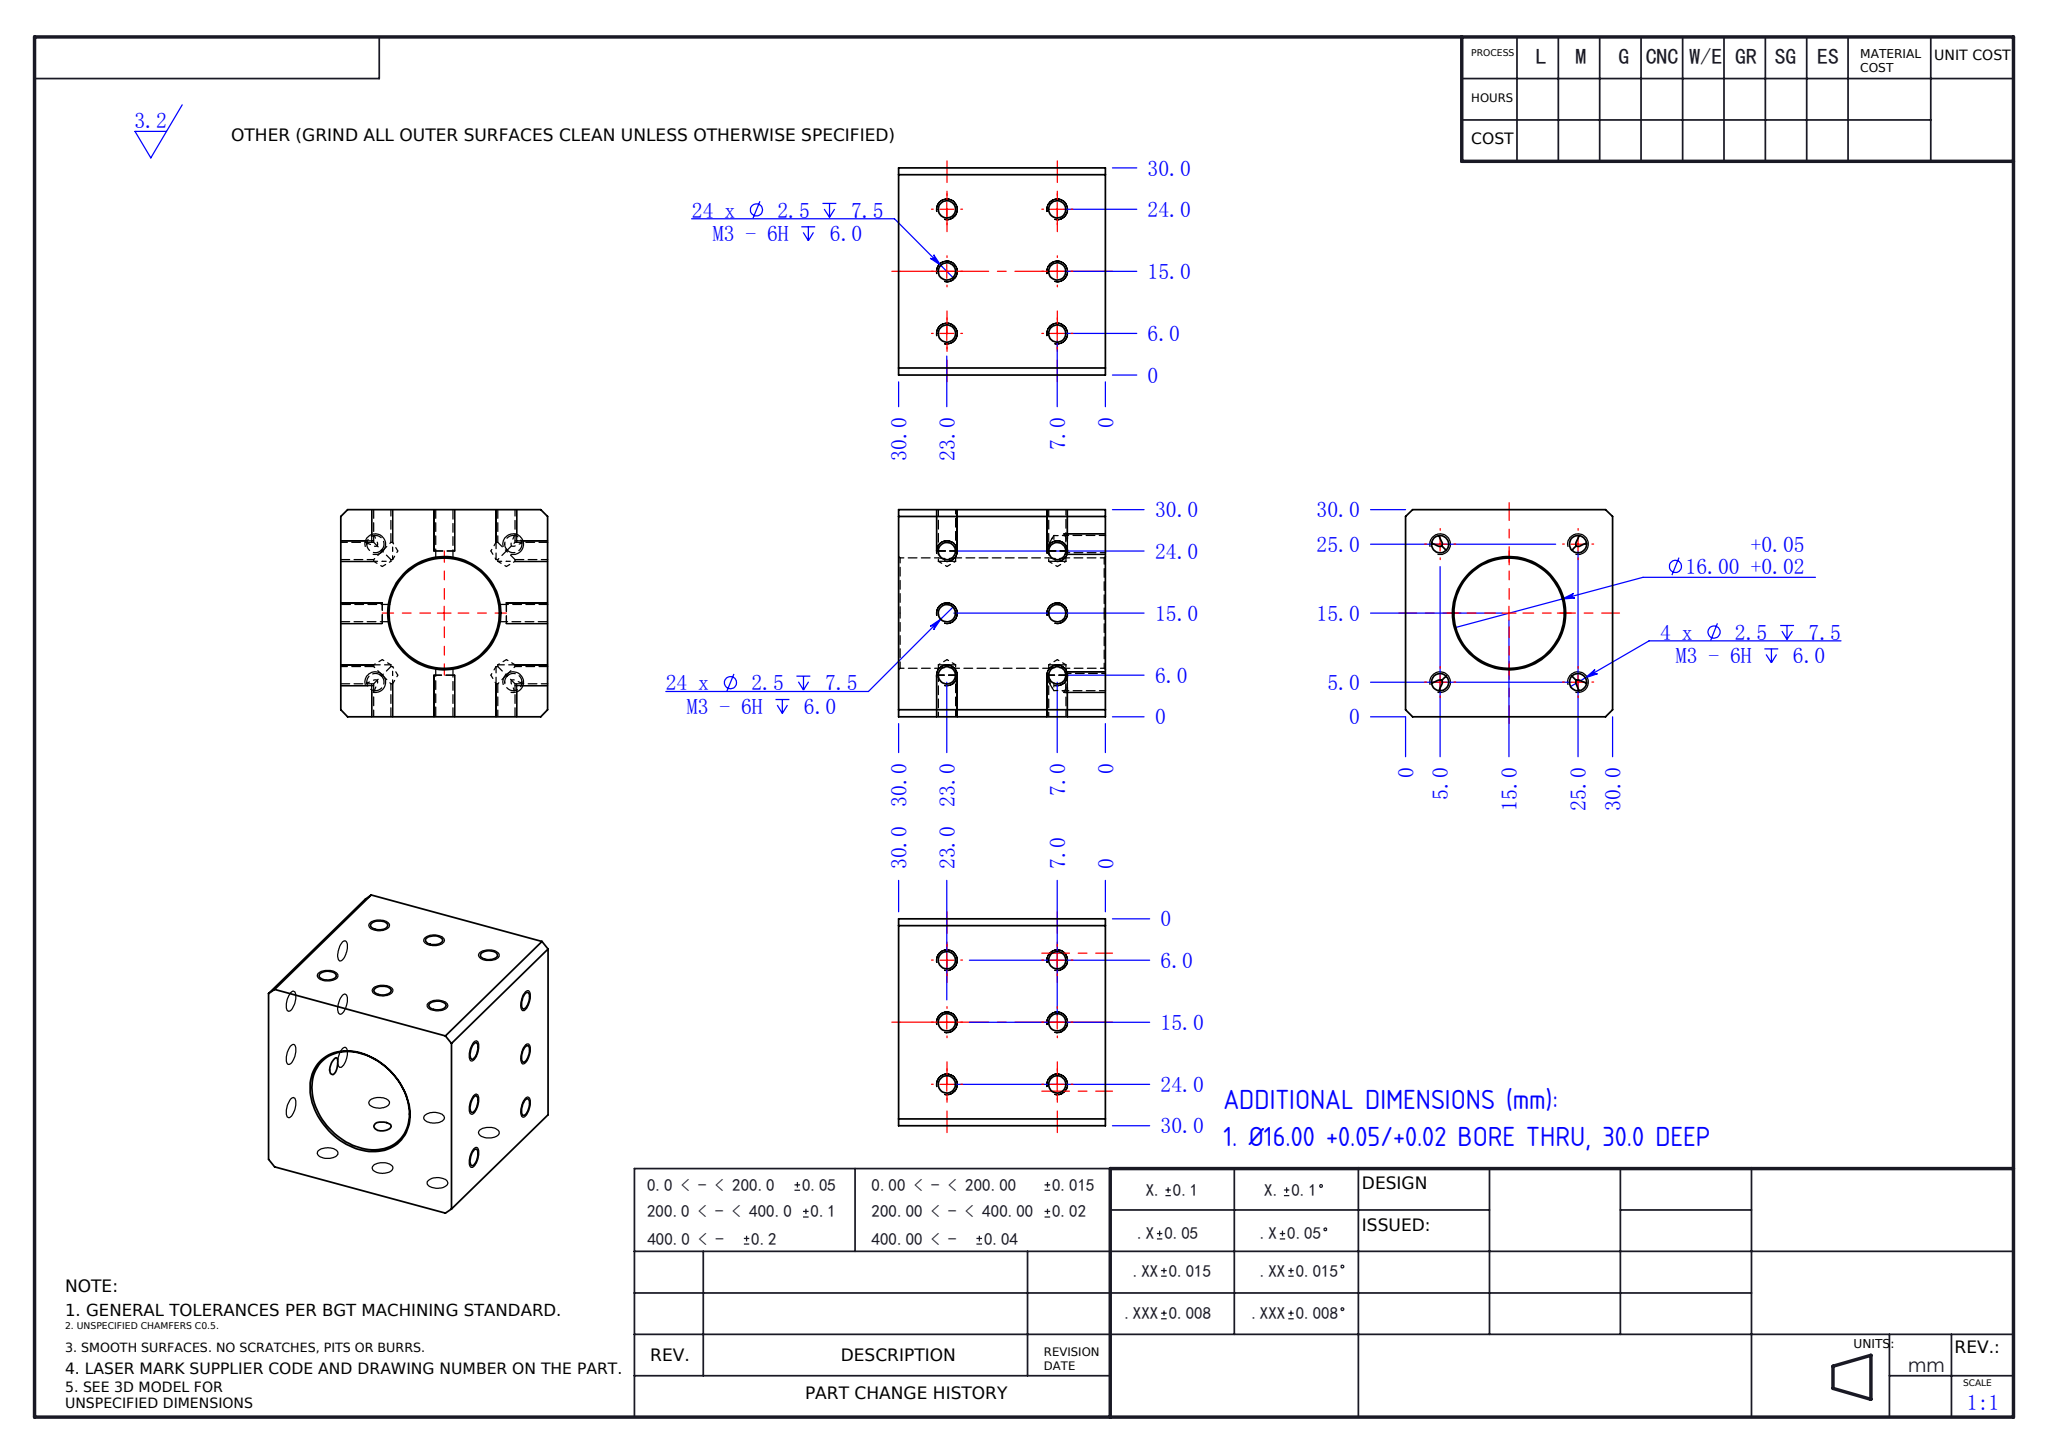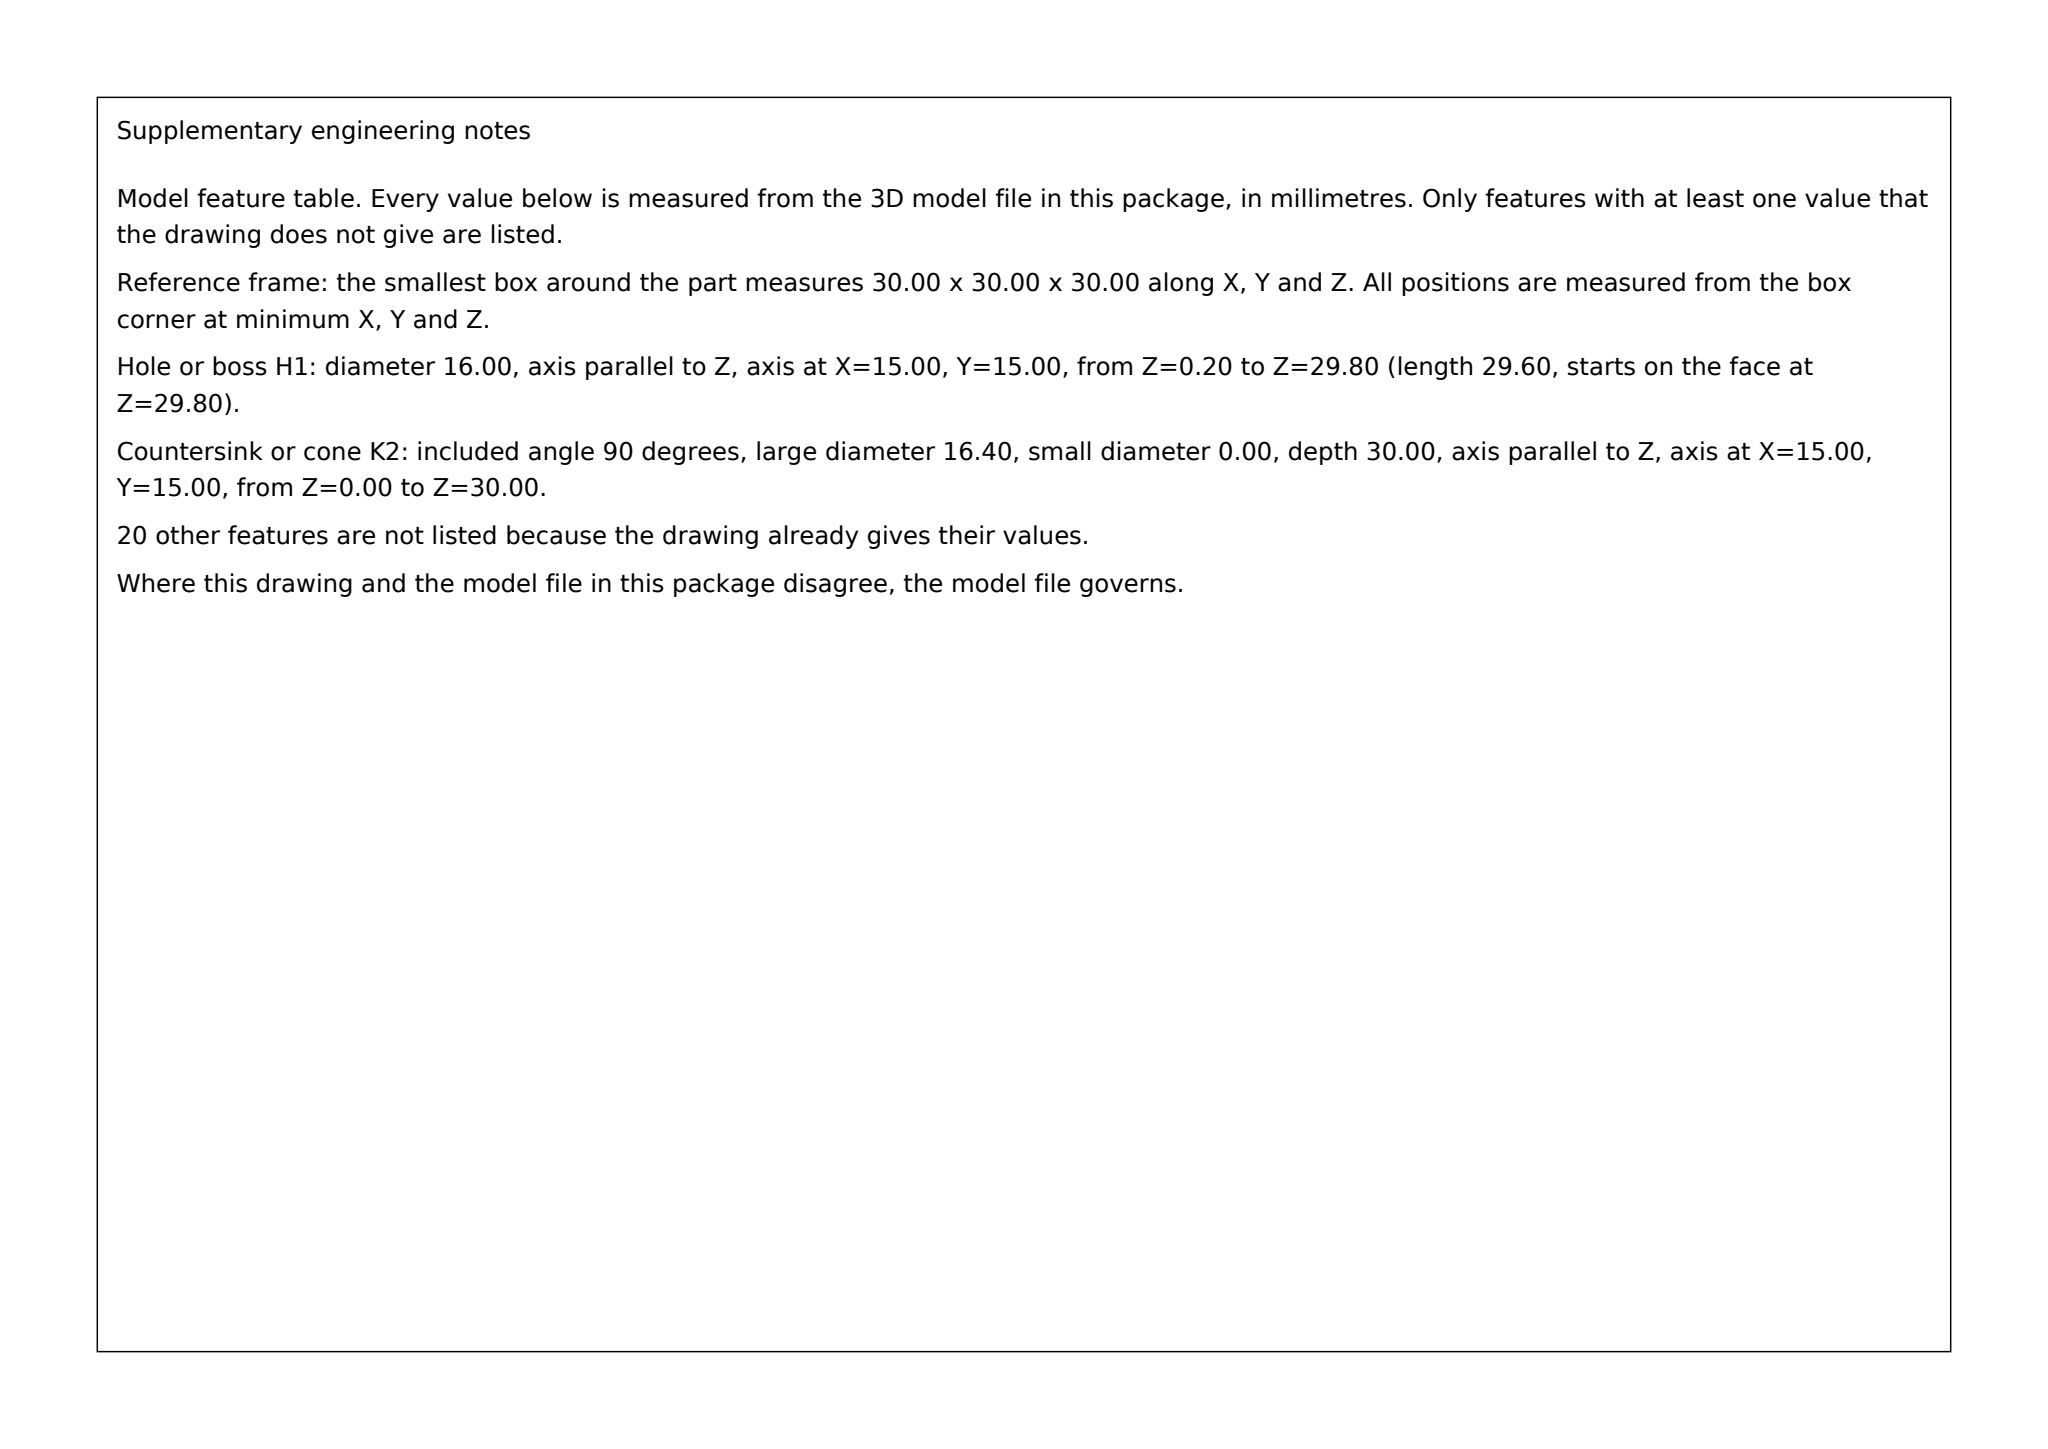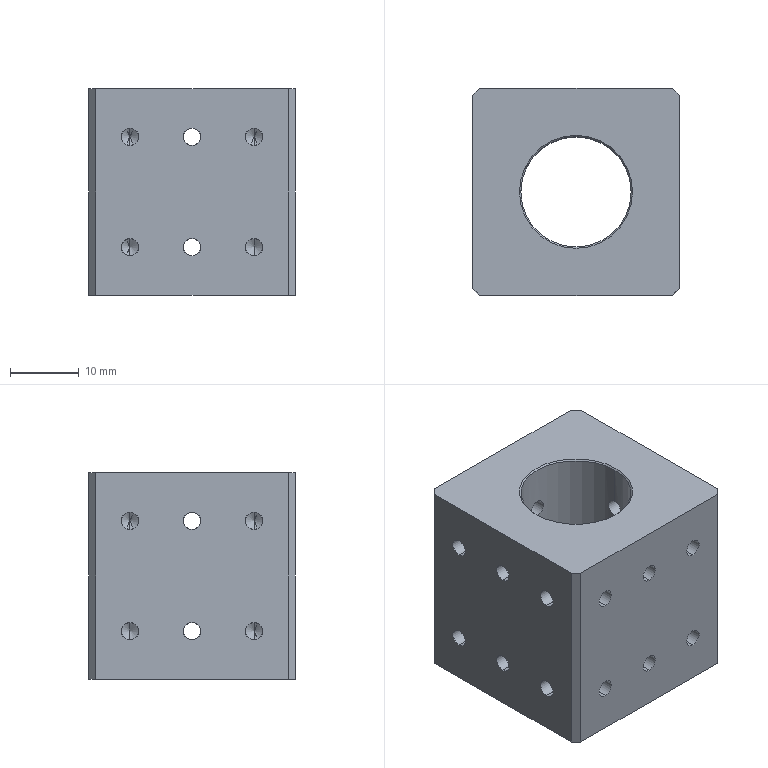Part | SolidWorks | mm | 1 solid | 152 faces | box 30 x 30 x 30 mm | volume 19982 mm3 | cylinder 98 | cone 44 | plane 10 | commonest cylinder face diameters 2.5 x96 16 x2
build123d program:
from build123d import *

# Parameters (mm, degrees)
SKETCH1_W                  = 30
SKETCH1_H                  = 30
SKETCH1_R                  = 8
BOSS_EXTRUDE1_DEPTH        = 30
M3_TAPPED_HOLE1_AT_2_COUNT = 2
M3_TAPPED_HOLE1_AT_2_PITCH = 16
M3_TAPPED_HOLE1_AT_3_COUNT = 2
M3_TAPPED_HOLE1_AT_3_PITCH = 18
M3_TAPPED_HOLE1_AT_4_COUNT = 2
M3_TAPPED_HOLE1_AT_4_PITCH = 24.083
M3_TAPPED_HOLE1_AT_5_COUNT = 2
M3_TAPPED_HOLE1_AT_5_PITCH = 9
M3_TAPPED_HOLE1_AT_6_COUNT = 2
M3_TAPPED_HOLE1_AT_6_PITCH = 18.358
CIRPATTERN1_COUNT          = 4
CHAMFER1_SIZE              = 1
M3_TAPPED_HOLE5_D          = 2.5
M3_TAPPED_HOLE5_DEPTH      = 7.5
M3_TAPPED_HOLE5_TIP        = 0.7511
CHAMFER2_SIZE              = 0.2


with BuildPart() as part:
    # Sketch1 → Boss-Extrude1 (new body)
    with BuildSketch(Plane.XY):
        Rectangle(SKETCH1_W, SKETCH1_H)
        Circle(SKETCH1_R, mode=Mode.SUBTRACT)
    extrude(amount=BOSS_EXTRUDE1_DEPTH)

    # Sketch3 → M3 Tapped Hole1 (revolve, cut)
    with BuildSketch(Plane(origin=(-9, 15, 7), x_dir=(0, 0, 1), z_dir=(1, 0, 0))):
        Polygon((0, 0), (0, 8.251), (1.25, 7.5), (1.25, 0), align=None)
    m3_tapped_hole1 = revolve(axis=Axis((-9, 21.35, 7), (0, -1, 0)), mode=Mode.SUBTRACT)

    # M3 Tapped Hole1 at 2: M3 Tapped Hole1 ×2
    with Locations(*[(0, 0, i * M3_TAPPED_HOLE1_AT_2_PITCH) for i in range(1, M3_TAPPED_HOLE1_AT_2_COUNT)]):
        add(m3_tapped_hole1, mode=Mode.SUBTRACT)

    # M3 Tapped Hole1 at 3: M3 Tapped Hole1 ×2
    with Locations(*[(i * M3_TAPPED_HOLE1_AT_3_PITCH, 0, 0) for i in range(1, M3_TAPPED_HOLE1_AT_3_COUNT)]):
        add(m3_tapped_hole1, mode=Mode.SUBTRACT)

    # M3 Tapped Hole1 at 4: M3 Tapped Hole1 ×2
    with Locations(*[Vector(0.7474, 0, 0.6644) * (i * M3_TAPPED_HOLE1_AT_4_PITCH) for i in range(1, M3_TAPPED_HOLE1_AT_4_COUNT)]):
        add(m3_tapped_hole1, mode=Mode.SUBTRACT)

    # M3 Tapped Hole1 at 5: M3 Tapped Hole1 ×2
    with Locations(*[(i * M3_TAPPED_HOLE1_AT_5_PITCH, 0, 0) for i in range(1, M3_TAPPED_HOLE1_AT_5_COUNT)]):
        add(m3_tapped_hole1, mode=Mode.SUBTRACT)

    # M3 Tapped Hole1 at 6: M3 Tapped Hole1 ×2
    with Locations(*[Vector(0.4903, 0, 0.8716) * (i * M3_TAPPED_HOLE1_AT_6_PITCH) for i in range(1, M3_TAPPED_HOLE1_AT_6_COUNT)]):
        add(m3_tapped_hole1, mode=Mode.SUBTRACT)

    # CirPattern1: M3 Tapped Hole1 ×4 about axis
    cirpattern1_axis = Axis((0, 0, 30), (0, 0, 1))
    for i in range(1, CIRPATTERN1_COUNT):
        add(m3_tapped_hole1.rotate(cirpattern1_axis, i * 360 / CIRPATTERN1_COUNT), mode=Mode.SUBTRACT)

    # CirPattern1 copy 1 sketch → CirPattern1 copy 1 (revolve, cut)
    with BuildSketch(Plane(origin=(-15, -9, 23), x_dir=(0, 0, 1), z_dir=(0, 1, 0))):
        Polygon((0, 0), (0, 8.251), (1.25, 7.5), (1.25, 0), align=None)
    revolve(axis=Axis((-21.35, -9, 23), (1, 0, 0)), mode=Mode.SUBTRACT)

    # CirPattern1 copy 2 sketch → CirPattern1 copy 2 (revolve, cut)
    with BuildSketch(Plane(origin=(9, -15, 23), x_dir=(0, 0, 1), z_dir=(-1, 0, 0))):
        Polygon((0, 0), (0, 8.251), (1.25, 7.5), (1.25, 0), align=None)
    revolve(axis=Axis((9, -21.35, 23), (0, 1, 0)), mode=Mode.SUBTRACT)

    # CirPattern1 copy 3 sketch → CirPattern1 copy 3 (revolve, cut)
    with BuildSketch(Plane(origin=(15, 9, 23), x_dir=(0, 0, 1), z_dir=(0, -1, 0))):
        Polygon((0, 0), (0, 8.251), (1.25, 7.5), (1.25, 0), align=None)
    revolve(axis=Axis((21.35, 9, 23), (-1, 0, 0)), mode=Mode.SUBTRACT)

    # CirPattern1 copy 4 sketch → CirPattern1 copy 4 (revolve, cut)
    with BuildSketch(Plane(origin=(-15, 9, 7), x_dir=(0, 0, 1), z_dir=(0, 1, 0))):
        Polygon((0, 0), (0, 8.251), (1.25, 7.5), (1.25, 0), align=None)
    revolve(axis=Axis((-21.35, 9, 7), (1, 0, 0)), mode=Mode.SUBTRACT)

    # CirPattern1 copy 5 sketch → CirPattern1 copy 5 (revolve, cut)
    with BuildSketch(Plane(origin=(-9, -15, 7), x_dir=(0, 0, 1), z_dir=(-1, 0, 0))):
        Polygon((0, 0), (0, 8.251), (1.25, 7.5), (1.25, 0), align=None)
    revolve(axis=Axis((-9, -21.35, 7), (0, 1, 0)), mode=Mode.SUBTRACT)

    # CirPattern1 copy 6 sketch → CirPattern1 copy 6 (revolve, cut)
    with BuildSketch(Plane(origin=(15, -9, 7), x_dir=(0, 0, 1), z_dir=(0, -1, 0))):
        Polygon((0, 0), (0, 8.251), (1.25, 7.5), (1.25, 0), align=None)
    revolve(axis=Axis((21.35, -9, 7), (-1, 0, 0)), mode=Mode.SUBTRACT)

    # CirPattern1 copy 7 sketch → CirPattern1 copy 7 (revolve, cut)
    with BuildSketch(Plane(origin=(-15, 9, 23), x_dir=(0, 0, 1), z_dir=(0, 1, 0))):
        Polygon((0, 0), (0, 8.251), (1.25, 7.5), (1.25, 0), align=None)
    revolve(axis=Axis((-21.35, 9, 23), (1, 0, 0)), mode=Mode.SUBTRACT)

    # CirPattern1 copy 8 sketch → CirPattern1 copy 8 (revolve, cut)
    with BuildSketch(Plane(origin=(-9, -15, 23), x_dir=(0, 0, 1), z_dir=(-1, 0, 0))):
        Polygon((0, 0), (0, 8.251), (1.25, 7.5), (1.25, 0), align=None)
    revolve(axis=Axis((-9, -21.35, 23), (0, 1, 0)), mode=Mode.SUBTRACT)

    # CirPattern1 copy 9 sketch → CirPattern1 copy 9 (revolve, cut)
    with BuildSketch(Plane(origin=(15, -9, 23), x_dir=(0, 0, 1), z_dir=(0, -1, 0))):
        Polygon((0, 0), (0, 8.251), (1.25, 7.5), (1.25, 0), align=None)
    revolve(axis=Axis((21.35, -9, 23), (-1, 0, 0)), mode=Mode.SUBTRACT)

    # CirPattern1 copy 10 sketch → CirPattern1 copy 10 (revolve, cut)
    with BuildSketch(Plane(origin=(-15, 0, 7), x_dir=(0, 0, 1), z_dir=(0, 1, 0))):
        Polygon((0, 0), (0, 8.251), (1.25, 7.5), (1.25, 0), align=None)
    revolve(axis=Axis((-21.35, 0, 7), (1, 0, 0)), mode=Mode.SUBTRACT)

    # CirPattern1 copy 11 sketch → CirPattern1 copy 11 (revolve, cut)
    with BuildSketch(Plane(origin=(0, -15, 7), x_dir=(0, 0, 1), z_dir=(-1, 0, 0))):
        Polygon((0, 0), (0, 8.251), (1.25, 7.5), (1.25, 0), align=None)
    revolve(axis=Axis((0, -21.35, 7), (0, 1, 0)), mode=Mode.SUBTRACT)

    # CirPattern1 copy 12 sketch → CirPattern1 copy 12 (revolve, cut)
    with BuildSketch(Plane(origin=(15, 0, 7), x_dir=(0, 0, 1), z_dir=(0, -1, 0))):
        Polygon((0, 0), (0, 8.251), (1.25, 7.5), (1.25, 0), align=None)
    revolve(axis=Axis((21.35, 0, 7), (-1, 0, 0)), mode=Mode.SUBTRACT)

    # CirPattern1 copy 13 sketch → CirPattern1 copy 13 (revolve, cut)
    with BuildSketch(Plane(origin=(-15, 0, 23), x_dir=(0, 0, 1), z_dir=(0, 1, 0))):
        Polygon((0, 0), (0, 8.251), (1.25, 7.5), (1.25, 0), align=None)
    revolve(axis=Axis((-21.35, 0, 23), (1, 0, 0)), mode=Mode.SUBTRACT)

    # CirPattern1 copy 14 sketch → CirPattern1 copy 14 (revolve, cut)
    with BuildSketch(Plane(origin=(0, -15, 23), x_dir=(0, 0, 1), z_dir=(-1, 0, 0))):
        Polygon((0, 0), (0, 8.251), (1.25, 7.5), (1.25, 0), align=None)
    revolve(axis=Axis((0, -21.35, 23), (0, 1, 0)), mode=Mode.SUBTRACT)

    # CirPattern1 copy 15 sketch → CirPattern1 copy 15 (revolve, cut)
    with BuildSketch(Plane(origin=(15, 0, 23), x_dir=(0, 0, 1), z_dir=(0, -1, 0))):
        Polygon((0, 0), (0, 8.251), (1.25, 7.5), (1.25, 0), align=None)
    revolve(axis=Axis((21.35, 0, 23), (-1, 0, 0)), mode=Mode.SUBTRACT)

    # Chamfer1
    chamfer1_edges = [part.edges().sort_by_distance(p)[0] for p in [
        (15, -15, 15),
        (-15, -15, 15),
        (-15, 15, 15),
        (15, 15, 15),
    ]]
    chamfer(chamfer1_edges, length=CHAMFER1_SIZE)

    # M3 Tapped Hole5
    with Locations(Plane(origin=(0, 0, 0), x_dir=(-1, 0, 0), z_dir=(0, 0, -1))):
        with Locations((10, 10), (10, -10), (-10, 10), (-10, -10)):
            Hole(M3_TAPPED_HOLE5_D / 2, depth=M3_TAPPED_HOLE5_DEPTH)
            with Locations((0, 0, -(M3_TAPPED_HOLE5_DEPTH + M3_TAPPED_HOLE5_TIP / 2))):  # 118° drill point
                Cone(0, M3_TAPPED_HOLE5_D / 2, M3_TAPPED_HOLE5_TIP, mode=Mode.SUBTRACT)

    # Chamfer2
    chamfer2_edges = [part.edges().sort_by_distance(p)[0] for p in [
        (-8, 0, 0),
        (-8, 0, 30),
    ]]
    chamfer(chamfer2_edges, length=CHAMFER2_SIZE)


solid = part.part